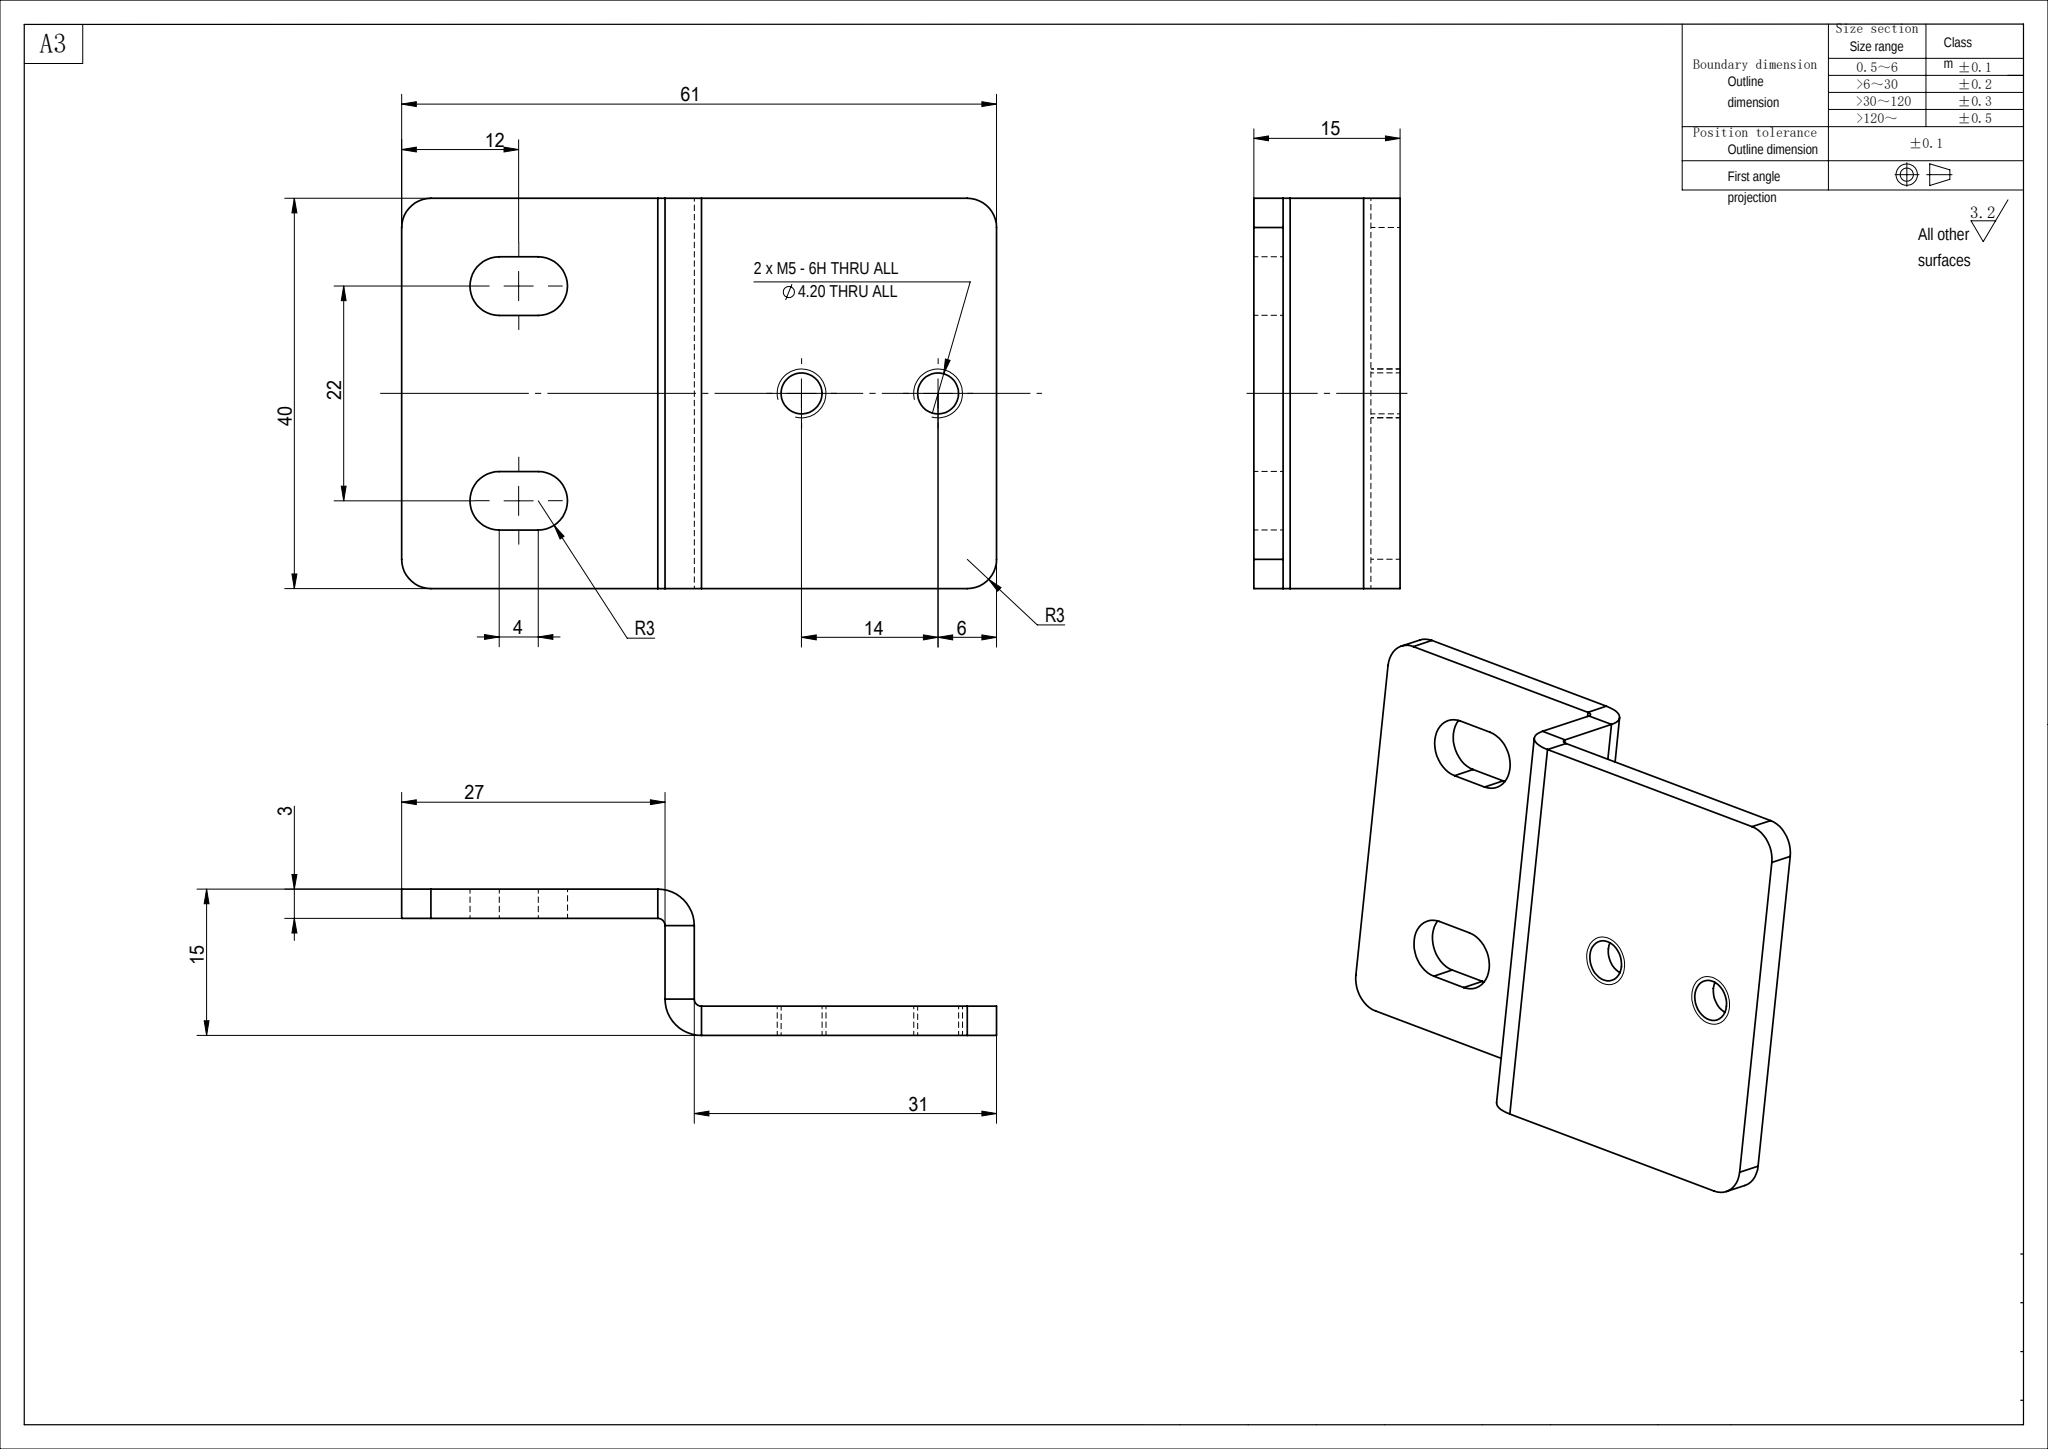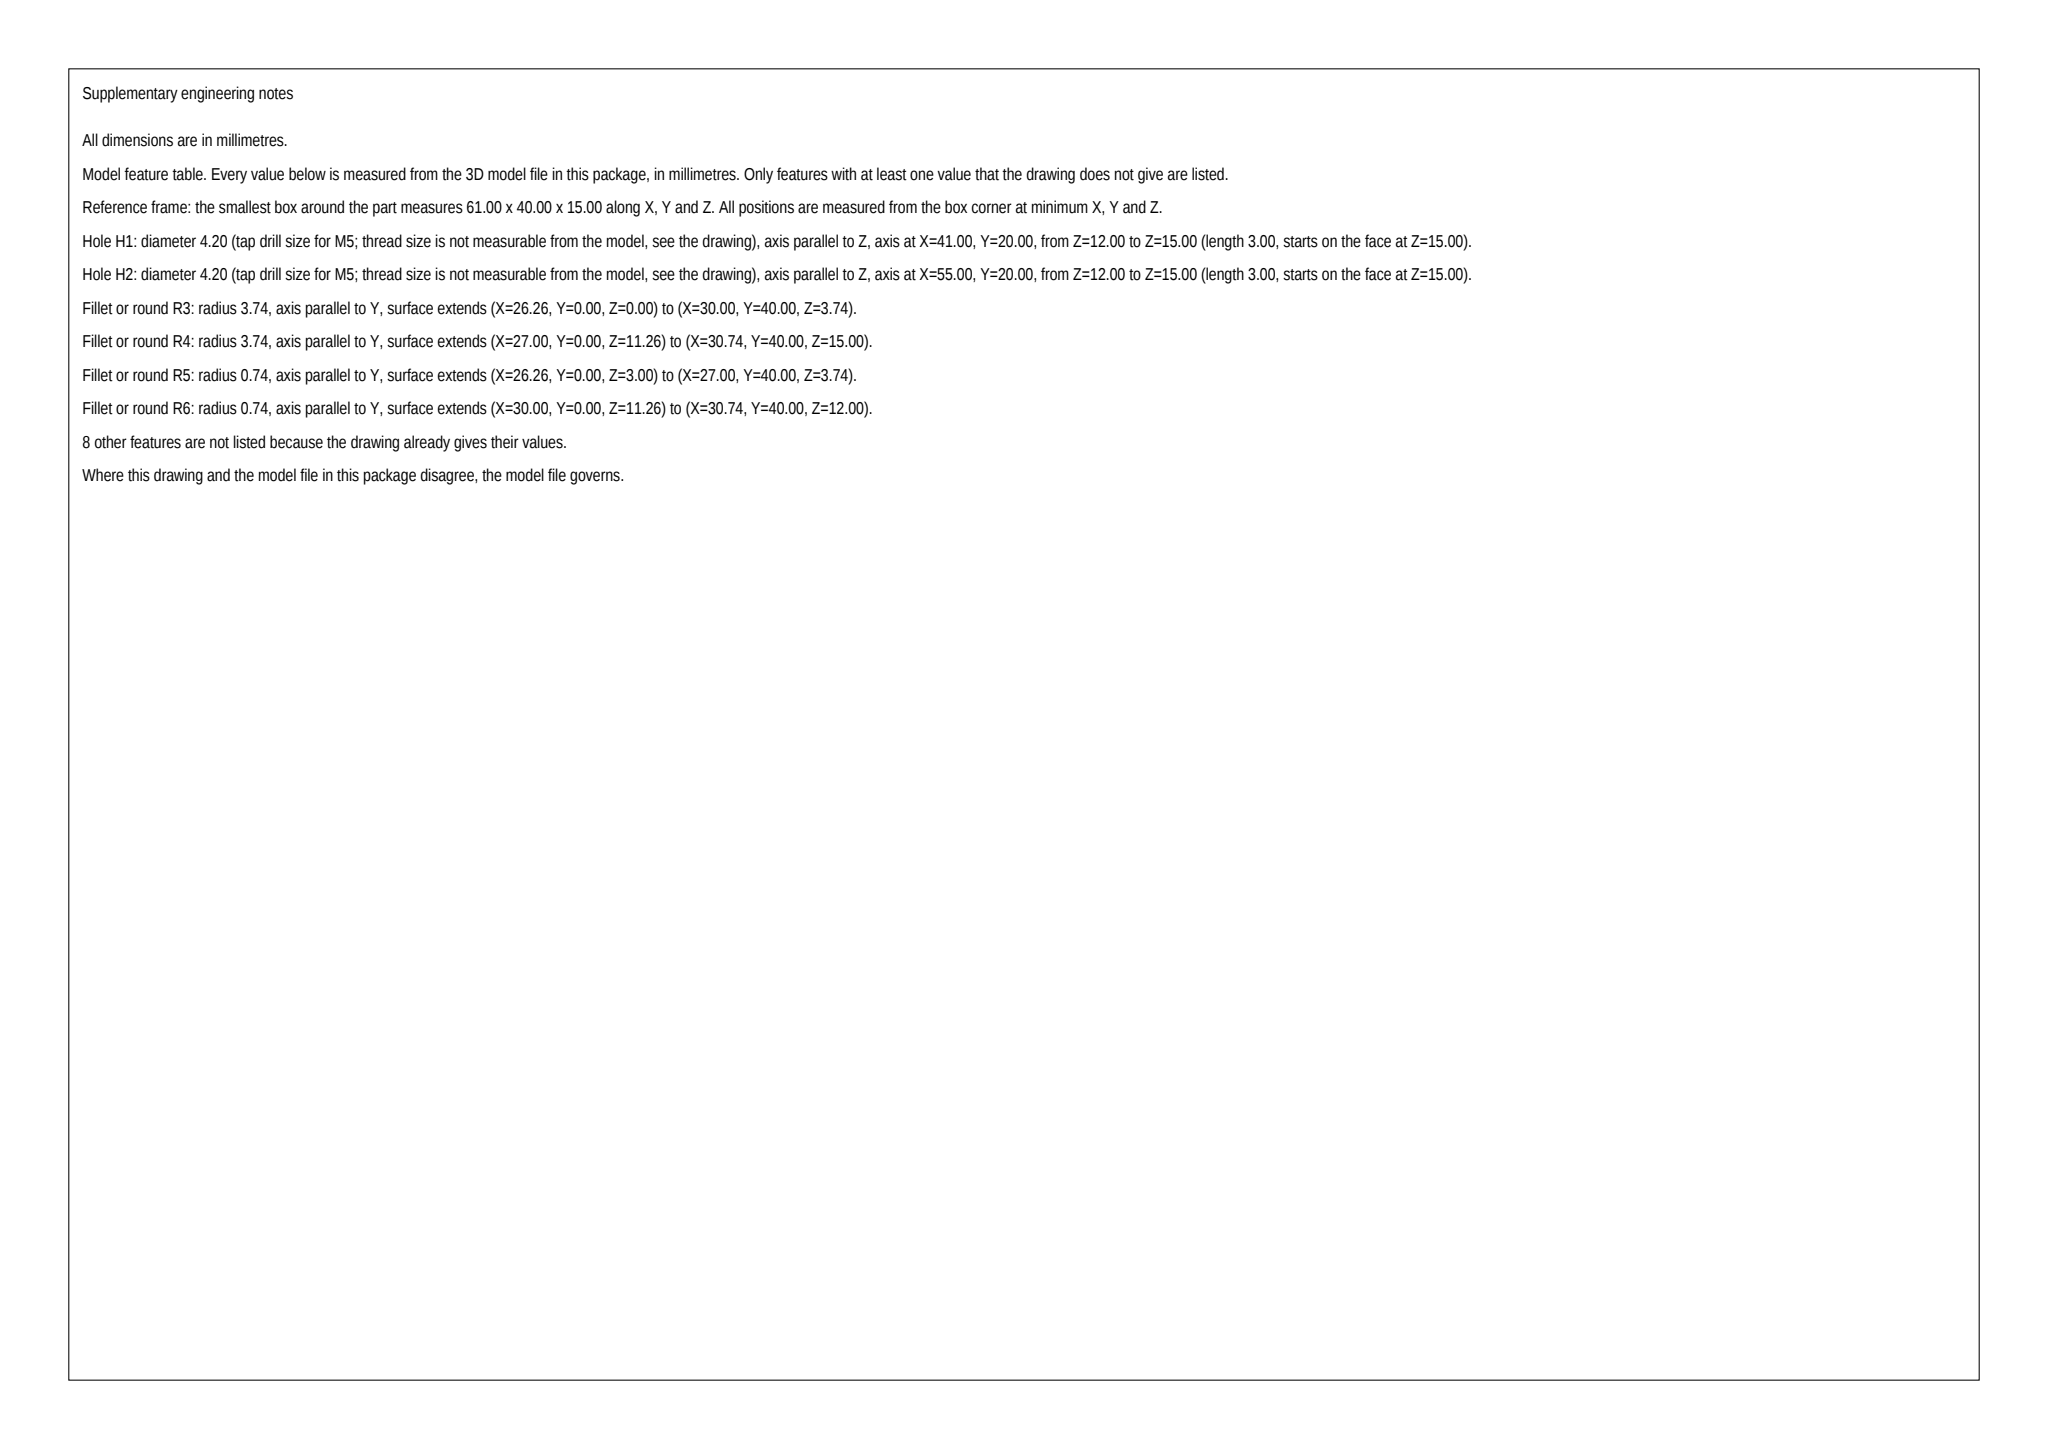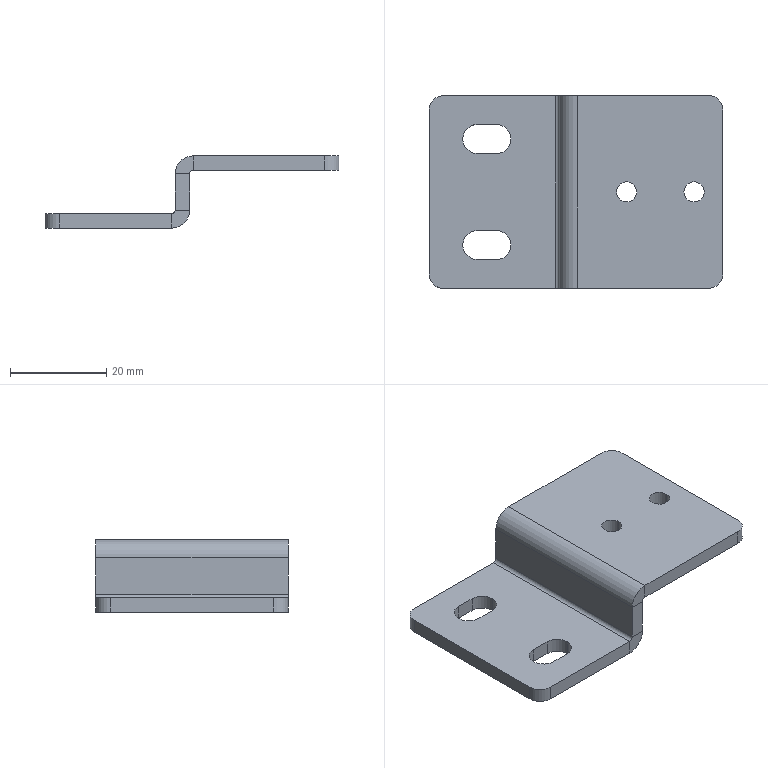Part | SolidWorks | mm | 1 solid | 40 faces | box 61 x 40 x 15 mm | volume 8110 mm3 | plane 22 | cylinder 18 | commonest cylinder face diameters 6 x10 4.2 x4 7.473 x2 1.473 x2